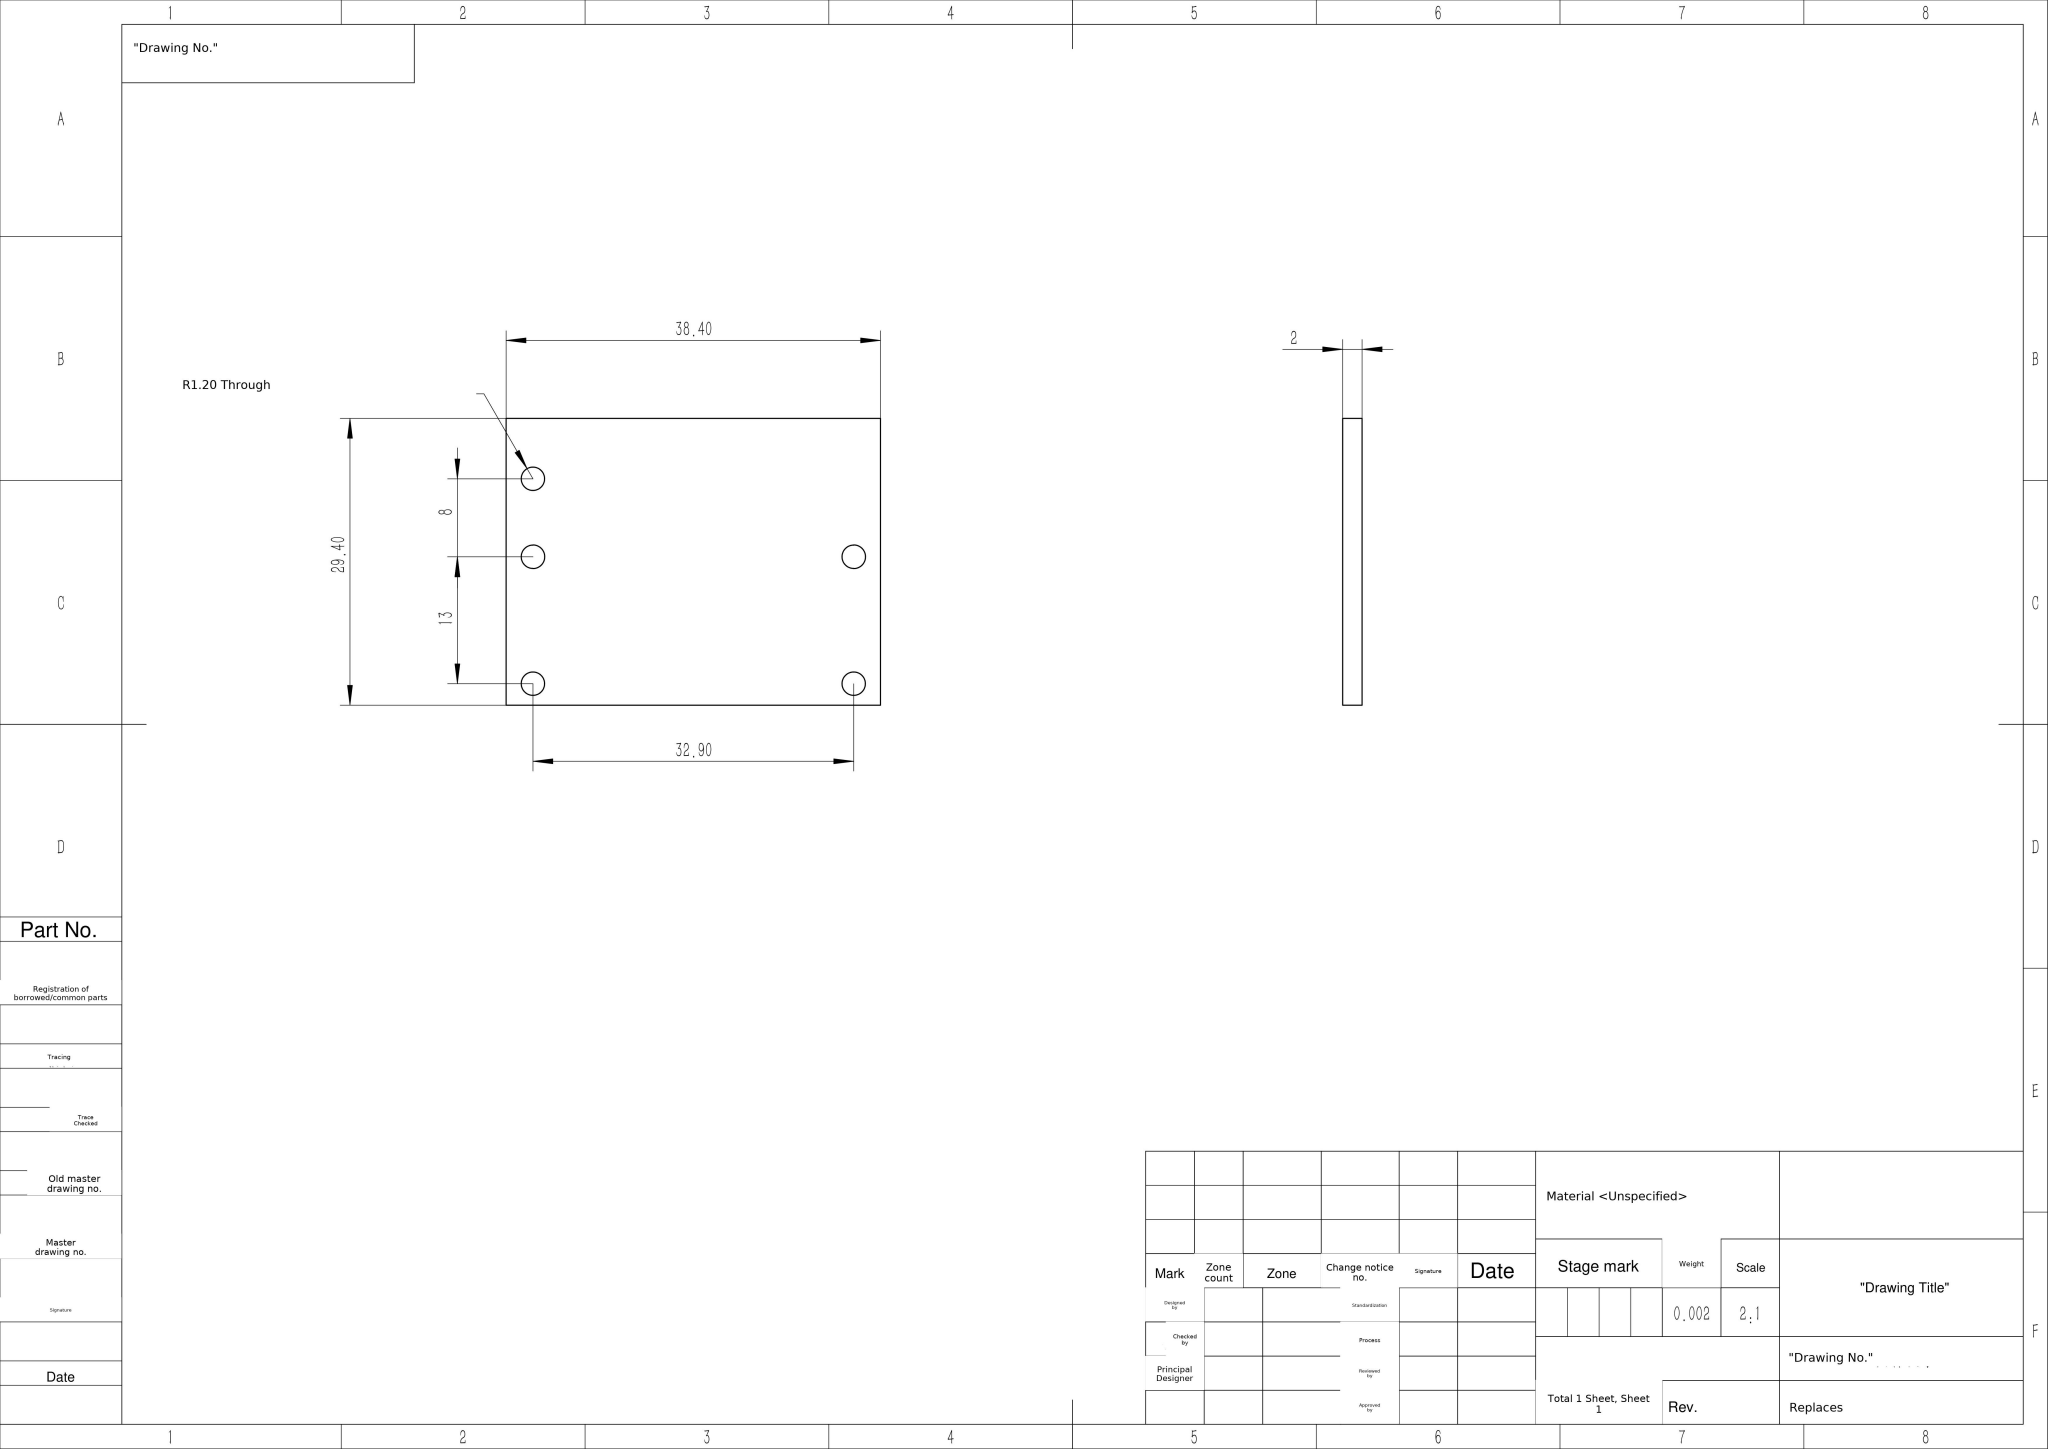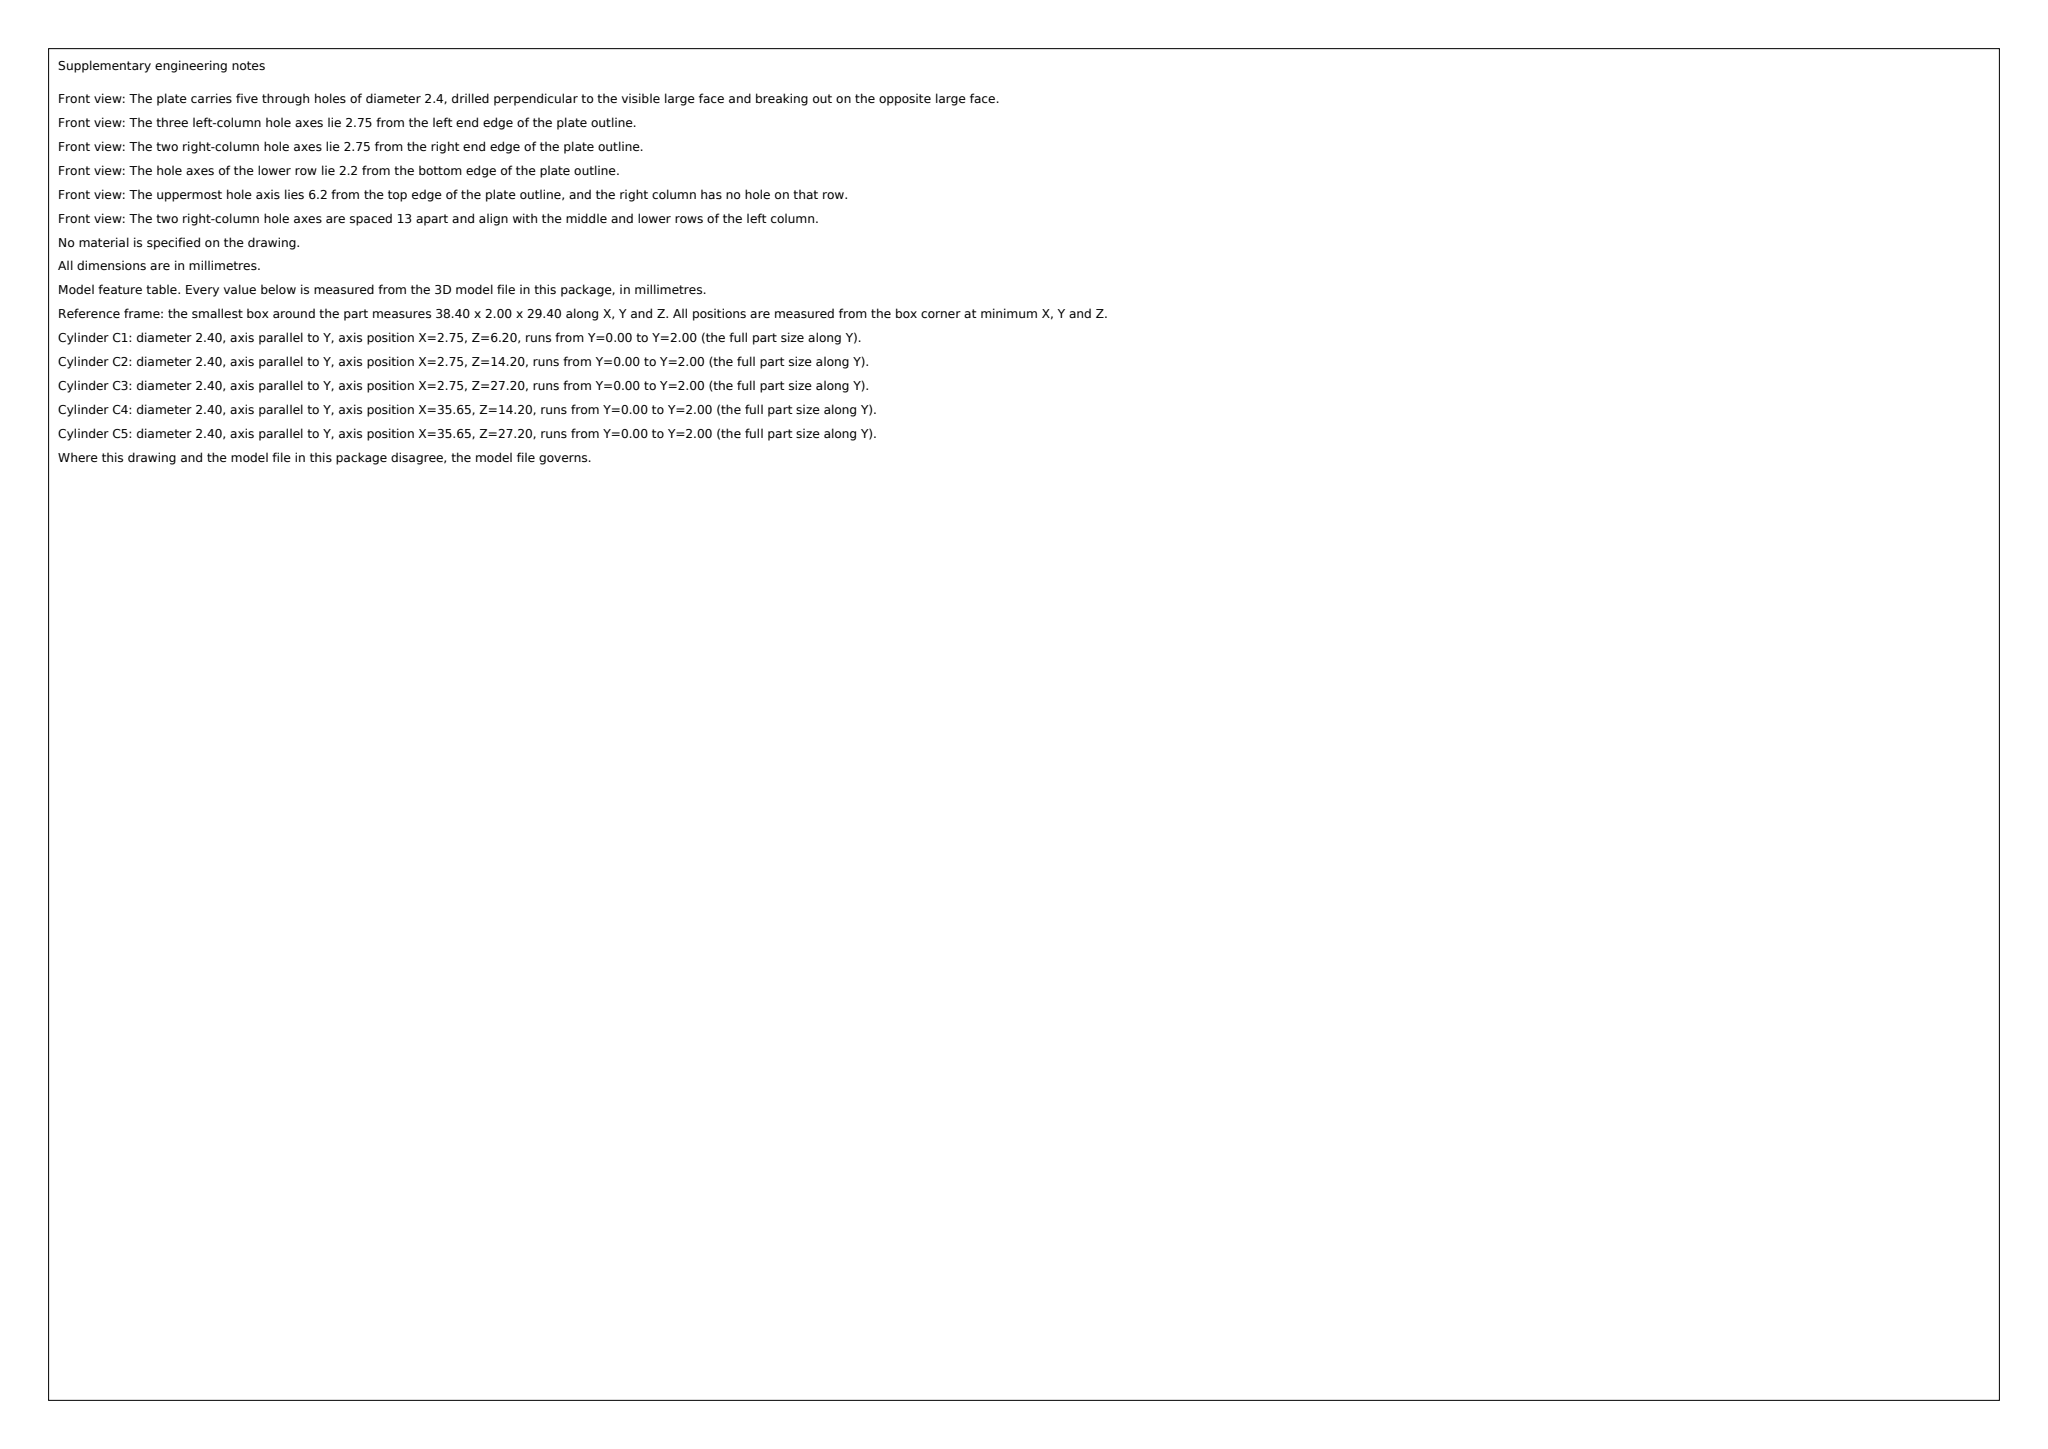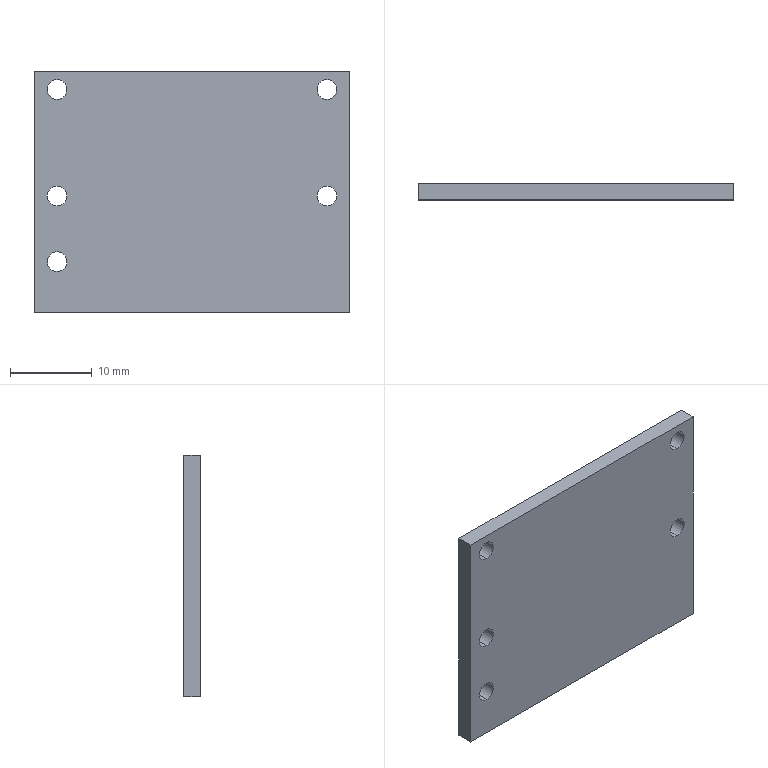Part | SolidWorks | mm | 1 solid | 16 faces | box 38.4 x 2 x 29.4 mm | volume 2213 mm3 | cylinder 10 | plane 6 | commonest cylinder face diameters 2.4 x10
Drawing notes:
TOP HOLE CL 2.2 FROM TOP EDGE; 8 & 13 TO LOWER HOLES | from the solid: Holes at z=27.2, 14.2, 6.2; plate height 29.4 -> 29.4-27.2=2.2
HOLE COL CL 2.75 FROM EA SIDE EDGE, 32.90 BETWEEN CL | from the solid: Hole x=2.75 and 35.65; bbox x=38.4 -> 38.4-35.65=2.75; 35.65-2.75=32.90
5X Ø2.4 THRU (R1.20) ALL HOLES | from the solid: Five cylinders dia 2.4, axis y, length 2.0 = full plate thickness 2.0
STEP:
#1=CARTESIAN_POINT('',(16.45,0.,-1.7));
#2=VERTEX_POINT('',#1);
#3=CARTESIAN_POINT('',(16.45,2.,-1.7));
#4=VERTEX_POINT('',#3);
#5=CARTESIAN_POINT('',(16.45,-0.001,-1.7));
#6=DIRECTION('',(0.,1.,0.));
#7=VECTOR('',#6,1000.);
#8=LINE('',#5,#7);
#9=EDGE_CURVE('',#2,#4,#8,.T.);
#10=ORIENTED_EDGE('',*,*,#9,.F.);
#11=CARTESIAN_POINT('',(16.45,0.,0.7));
#12=VERTEX_POINT('',#11);
#13=CARTESIAN_POINT('',(16.45,0.,-0.5));
#14=DIRECTION('',(0.,-1.,0.));
#15=DIRECTION('',(0.,0.,1.));
#16=AXIS2_PLACEMENT_3D('',#13,#14,#15);
#17=CIRCLE('',#16,1.2);
#18=EDGE_CURVE('',#2,#12,#17,.T.);
#19=ORIENTED_EDGE('',*,*,#18,.T.);
#20=CARTESIAN_POINT('',(16.45,2.,0.7));
#21=VERTEX_POINT('',#20);
#22=CARTESIAN_POINT('',(16.45,-0.001,0.7));
#23=DIRECTION('',(0.,1.,0.));
#24=VECTOR('',#23,1000.);
#25=LINE('',#22,#24);
#26=EDGE_CURVE('',#12,#21,#25,.T.);
#27=ORIENTED_EDGE('',*,*,#26,.T.);
#28=CARTESIAN_POINT('',(16.45,2.,-0.5));
#29=DIRECTION('',(0.,1.,0.));
#30=DIRECTION('',(0.,0.,1.));
#31=AXIS2_PLACEMENT_3D('',#28,#29,#30);
#32=CIRCLE('',#31,1.2);
#33=EDGE_CURVE('',#21,#4,#32,.T.);
#34=ORIENTED_EDGE('',*,*,#33,.T.);
#35=EDGE_LOOP('',(#10,#19,#27,#34));
#36=FACE_OUTER_BOUND('',#35,.T.);
#37=CARTESIAN_POINT('',(16.45,-0.001,-0.5));
#38=DIRECTION('',(0.,1.,0.));
#39=DIRECTION('',(0.,0.,1.));
#40=AXIS2_PLACEMENT_3D('',#37,#38,#39);
#41=CYLINDRICAL_SURFACE('',#40,1.2);
#42=ADVANCED_FACE('',(#36),#41,.F.);
#43=CARTESIAN_POINT('',(-16.45,0.,11.3));
#44=VERTEX_POINT('',#43);
#45=CARTESIAN_POINT('',(-16.45,2.,11.3));
#46=VERTEX_POINT('',#45);
#47=CARTESIAN_POINT('',(-16.45,-0.001,11.3));
#48=DIRECTION('',(0.,1.,0.));
#49=VECTOR('',#48,1000.);
#50=LINE('',#47,#49);
#51=EDGE_CURVE('',#44,#46,#50,.T.);
#52=ORIENTED_EDGE('',*,*,#51,.F.);
#53=CARTESIAN_POINT('',(-16.45,0.,13.7));
#54=VERTEX_POINT('',#53);
#55=CARTESIAN_POINT('',(-16.45,0.,12.5));
#56=DIRECTION('',(0.,-1.,0.));
#57=DIRECTION('',(0.,0.,1.));
#58=AXIS2_PLACEMENT_3D('',#55,#56,#57);
#59=CIRCLE('',#58,1.2);
#60=EDGE_CURVE('',#44,#54,#59,.T.);
#61=ORIENTED_EDGE('',*,*,#60,.T.);
#62=CARTESIAN_POINT('',(-16.45,2.,13.7));
#63=VERTEX_POINT('',#62);
#64=CARTESIAN_POINT('',(-16.45,-0.001,13.7));
#65=DIRECTION('',(0.,1.,0.));
#66=VECTOR('',#65,1000.);
#67=LINE('',#64,#66);
#68=EDGE_CURVE('',#54,#63,#67,.T.);
#69=ORIENTED_EDGE('',*,*,#68,.T.);
#70=CARTESIAN_POINT('',(-16.45,2.,12.5));
#71=DIRECTION('',(0.,1.,0.));
#72=DIRECTION('',(0.,0.,1.));
#73=AXIS2_PLACEMENT_3D('',#70,#71,#72);
#74=CIRCLE('',#73,1.2);
#75=EDGE_CURVE('',#63,#46,#74,.T.);
#76=ORIENTED_EDGE('',*,*,#75,.T.);
#77=EDGE_LOOP('',(#52,#61,#69,#76));
#78=FACE_OUTER_BOUND('',#77,.T.);
#79=CARTESIAN_POINT('',(-16.45,-0.001,12.5));
#80=DIRECTION('',(0.,1.,0.));
#81=DIRECTION('',(0.,0.,1.));
#82=AXIS2_PLACEMENT_3D('',#79,#80,#81);
#83=CYLINDRICAL_SURFACE('',#82,1.2);
#84=ADVANCED_FACE('',(#78),#83,.F.);
#85=CARTESIAN_POINT('',(-16.45,0.,-1.7));
#86=VERTEX_POINT('',#85);
#87=CARTESIAN_POINT('',(-16.45,2.,-1.7));
#88=VERTEX_POINT('',#87);
#89=CARTESIAN_POINT('',(-16.45,-0.001,-1.7));
#90=DIRECTION('',(0.,1.,0.));
#91=VECTOR('',#90,1000.);
#92=LINE('',#89,#91);
#93=EDGE_CURVE('',#86,#88,#92,.T.);
#94=ORIENTED_EDGE('',*,*,#93,.F.);
#95=CARTESIAN_POINT('',(-16.45,0.,0.7));
#96=VERTEX_POINT('',#95);
#97=CARTESIAN_POINT('',(-16.45,0.,-0.5));
#98=DIRECTION('',(0.,-1.,0.));
#99=DIRECTION('',(0.,0.,1.));
#100=AXIS2_PLACEMENT_3D('',#97,#98,#99);
#101=CIRCLE('',#100,1.2);
#102=EDGE_CURVE('',#86,#96,#101,.T.);
#103=ORIENTED_EDGE('',*,*,#102,.T.);
#104=CARTESIAN_POINT('',(-16.45,2.,0.7));
#105=VERTEX_POINT('',#104);
#106=CARTESIAN_POINT('',(-16.45,-0.001,0.7));
#107=DIRECTION('',(0.,1.,0.));
#108=VECTOR('',#107,1000.);
#109=LINE('',#106,#108);
#110=EDGE_CURVE('',#96,#105,#109,.T.);
#111=ORIENTED_EDGE('',*,*,#110,.T.);
#112=CARTESIAN_POINT('',(-16.45,2.,-0.5));
#113=DIRECTION('',(0.,1.,0.));
#114=DIRECTION('',(0.,0.,1.));
#115=AXIS2_PLACEMENT_3D('',#112,#113,#114);
#116=CIRCLE('',#115,1.2);
#117=EDGE_CURVE('',#105,#88,#116,.T.);
#118=ORIENTED_EDGE('',*,*,#117,.T.);
#119=EDGE_LOOP('',(#94,#103,#111,#118));
#120=FACE_OUTER_BOUND('',#119,.T.);
#121=CARTESIAN_POINT('',(-16.45,-0.001,-0.5));
#122=DIRECTION('',(0.,1.,0.));
#123=DIRECTION('',(0.,0.,1.));
#124=AXIS2_PLACEMENT_3D('',#121,#122,#123);
#125=CYLINDRICAL_SURFACE('',#124,1.2);
#126=ADVANCED_FACE('',(#120),#125,.F.);
#127=CARTESIAN_POINT('',(-16.45,0.,-9.7));
#128=VERTEX_POINT('',#127);
#129=CARTESIAN_POINT('',(-16.45,2.,-9.7));
#130=VERTEX_POINT('',#129);
#131=CARTESIAN_POINT('',(-16.45,-0.001,-9.7));
#132=DIRECTION('',(0.,1.,0.));
#133=VECTOR('',#132,1000.);
#134=LINE('',#131,#133);
#135=EDGE_CURVE('',#128,#130,#134,.T.);
#136=ORIENTED_EDGE('',*,*,#135,.F.);
#137=CARTESIAN_POINT('',(-16.45,0.,-7.3));
#138=VERTEX_POINT('',#137);
#139=CARTESIAN_POINT('',(-16.45,0.,-8.5));
#140=DIRECTION('',(0.,-1.,0.));
#141=DIRECTION('',(0.,0.,1.));
#142=AXIS2_PLACEMENT_3D('',#139,#140,#141);
#143=CIRCLE('',#142,1.2);
#144=EDGE_CURVE('',#128,#138,#143,.T.);
#145=ORIENTED_EDGE('',*,*,#144,.T.);
#146=CARTESIAN_POINT('',(-16.45,2.,-7.3));
#147=VERTEX_POINT('',#146);
#148=CARTESIAN_POINT('',(-16.45,-0.001,-7.3));
#149=DIRECTION('',(0.,1.,0.));
#150=VECTOR('',#149,1000.);
#151=LINE('',#148,#150);
#152=EDGE_CURVE('',#138,#147,#151,.T.);
#153=ORIENTED_EDGE('',*,*,#152,.T.);
#154=CARTESIAN_POINT('',(-16.45,2.,-8.5));
#155=DIRECTION('',(0.,1.,0.));
#156=DIRECTION('',(0.,0.,1.));
#157=AXIS2_PLACEMENT_3D('',#154,#155,#156);
#158=CIRCLE('',#157,1.2);
#159=EDGE_CURVE('',#147,#130,#158,.T.);
#160=ORIENTED_EDGE('',*,*,#159,.T.);
#161=EDGE_LOOP('',(#136,#145,#153,#160));
#162=FACE_OUTER_BOUND('',#161,.T.);
#163=CARTESIAN_POINT('',(-16.45,-0.001,-8.5));
#164=DIRECTION('',(0.,1.,0.));
#165=DIRECTION('',(0.,0.,1.));
#166=AXIS2_PLACEMENT_3D('',#163,#164,#165);
#167=CYLINDRICAL_SURFACE('',#166,1.2);
#168=ADVANCED_FACE('',(#162),#167,.F.);
#169=CARTESIAN_POINT('',(16.45,0.,11.3));
#170=VERTEX_POINT('',#169);
#171=CARTESIAN_POINT('',(16.45,2.,11.3));
#172=VERTEX_POINT('',#171);
#173=CARTESIAN_POINT('',(16.45,-0.001,11.3));
#174=DIRECTION('',(0.,1.,0.));
#175=VECTOR('',#174,1000.);
#176=LINE('',#173,#175);
#177=EDGE_CURVE('',#170,#172,#176,.T.);
#178=ORIENTED_EDGE('',*,*,#177,.F.);
#179=CARTESIAN_POINT('',(16.45,0.,13.7));
#180=VERTEX_POINT('',#179);
#181=CARTESIAN_POINT('',(16.45,0.,12.5));
#182=DIRECTION('',(0.,-1.,0.));
#183=DIRECTION('',(0.,0.,1.));
#184=AXIS2_PLACEMENT_3D('',#181,#182,#183);
#185=CIRCLE('',#184,1.2);
#186=EDGE_CURVE('',#170,#180,#185,.T.);
#187=ORIENTED_EDGE('',*,*,#186,.T.);
#188=CARTESIAN_POINT('',(16.45,2.,13.7));
#189=VERTEX_POINT('',#188);
#190=CARTESIAN_POINT('',(16.45,-0.001,13.7));
#191=DIRECTION('',(0.,1.,0.));
#192=VECTOR('',#191,1000.);
#193=LINE('',#190,#192);
#194=EDGE_CURVE('',#180,#189,#193,.T.);
#195=ORIENTED_EDGE('',*,*,#194,.T.);
#196=CARTESIAN_POINT('',(16.45,2.,12.5));
#197=DIRECTION('',(0.,1.,0.));
#198=DIRECTION('',(0.,0.,1.));
#199=AXIS2_PLACEMENT_3D('',#196,#197,#198);
#200=CIRCLE('',#199,1.2);
#201=EDGE_CURVE('',#189,#172,#200,.T.);
#202=ORIENTED_EDGE('',*,*,#201,.T.);
#203=EDGE_LOOP('',(#178,#187,#195,#202));
#204=FACE_OUTER_BOUND('',#203,.T.);
#205=CARTESIAN_POINT('',(16.45,-0.001,12.5));
#206=DIRECTION('',(0.,1.,0.));
#207=DIRECTION('',(0.,0.,1.));
#208=AXIS2_PLACEMENT_3D('',#205,#206,#207);
#209=CYLINDRICAL_SURFACE('',#208,1.2);
#210=ADVANCED_FACE('',(#204),#209,.F.);
#211=CARTESIAN_POINT('',(16.45,0.,12.5));
#212=DIRECTION('',(0.,-1.,0.));
#213=DIRECTION('',(0.,0.,1.));
#214=AXIS2_PLACEMENT_3D('',#211,#212,#213);
#215=CIRCLE('',#214,1.2);
#216=EDGE_CURVE('',#180,#170,#215,.T.);
#217=ORIENTED_EDGE('',*,*,#216,.F.);
#218=ORIENTED_EDGE('',*,*,#186,.F.);
#219=EDGE_LOOP('',(#217,#218));
#220=FACE_BOUND('',#219,.T.);
#221=CARTESIAN_POINT('',(-16.45,0.,-8.5));
#222=DIRECTION('',(0.,-1.,0.));
#223=DIRECTION('',(0.,0.,1.));
#224=AXIS2_PLACEMENT_3D('',#221,#222,#223);
#225=CIRCLE('',#224,1.2);
#226=EDGE_CURVE('',#138,#128,#225,.T.);
#227=ORIENTED_EDGE('',*,*,#226,.F.);
#228=ORIENTED_EDGE('',*,*,#144,.F.);
#229=EDGE_LOOP('',(#227,#228));
#230=FACE_BOUND('',#229,.T.);
#231=CARTESIAN_POINT('',(-16.45,0.,-0.5));
#232=DIRECTION('',(0.,-1.,0.));
#233=DIRECTION('',(0.,0.,1.));
#234=AXIS2_PLACEMENT_3D('',#231,#232,#233);
#235=CIRCLE('',#234,1.2);
#236=EDGE_CURVE('',#96,#86,#235,.T.);
#237=ORIENTED_EDGE('',*,*,#236,.F.);
#238=ORIENTED_EDGE('',*,*,#102,.F.);
#239=EDGE_LOOP('',(#237,#238));
#240=FACE_BOUND('',#239,.T.);
#241=CARTESIAN_POINT('',(-16.45,0.,12.5));
#242=DIRECTION('',(0.,-1.,0.));
#243=DIRECTION('',(0.,0.,1.));
#244=AXIS2_PLACEMENT_3D('',#241,#242,#243);
#245=CIRCLE('',#244,1.2);
#246=EDGE_CURVE('',#54,#44,#245,.T.);
#247=ORIENTED_EDGE('',*,*,#246,.F.);
#248=ORIENTED_EDGE('',*,*,#60,.F.);
#249=EDGE_LOOP('',(#247,#248));
#250=FACE_BOUND('',#249,.T.);
#251=CARTESIAN_POINT('',(16.45,0.,-0.5));
#252=DIRECTION('',(0.,-1.,0.));
#253=DIRECTION('',(0.,0.,1.));
#254=AXIS2_PLACEMENT_3D('',#251,#252,#253);
#255=CIRCLE('',#254,1.2);
#256=EDGE_CURVE('',#12,#2,#255,.T.);
#257=ORIENTED_EDGE('',*,*,#256,.F.);
#258=ORIENTED_EDGE('',*,*,#18,.F.);
#259=EDGE_LOOP('',(#257,#258));
#260=FACE_BOUND('',#259,.T.);
#261=CARTESIAN_POINT('',(19.2,0.,14.7));
#262=VERTEX_POINT('',#261);
#263=CARTESIAN_POINT('',(19.2,0.,-14.7));
#264=VERTEX_POINT('',#263);
#265=CARTESIAN_POINT('',(19.2,0.,-14.7));
#266=DIRECTION('',(0.,0.,-1.));
#267=VECTOR('',#266,1000.);
#268=LINE('',#265,#267);
#269=EDGE_CURVE('',#262,#264,#268,.T.);
#270=ORIENTED_EDGE('',*,*,#269,.F.);
#271=CARTESIAN_POINT('',(-19.2,0.,14.7));
#272=VERTEX_POINT('',#271);
#273=CARTESIAN_POINT('',(-19.2,0.,14.7));
#274=DIRECTION('',(1.,0.,0.));
#275=VECTOR('',#274,1000.);
#276=LINE('',#273,#275);
#277=EDGE_CURVE('',#272,#262,#276,.T.);
#278=ORIENTED_EDGE('',*,*,#277,.F.);
#279=CARTESIAN_POINT('',(-19.2,0.,-14.7));
#280=VERTEX_POINT('',#279);
#281=CARTESIAN_POINT('',(-19.2,0.,-14.7));
#282=DIRECTION('',(0.,0.,1.));
#283=VECTOR('',#282,1000.);
#284=LINE('',#281,#283);
#285=EDGE_CURVE('',#280,#272,#284,.T.);
#286=ORIENTED_EDGE('',*,*,#285,.F.);
#287=CARTESIAN_POINT('',(-19.2,0.,-14.7));
#288=DIRECTION('',(-1.,0.,0.));
#289=VECTOR('',#288,1000.);
#290=LINE('',#287,#289);
#291=EDGE_CURVE('',#264,#280,#290,.T.);
#292=ORIENTED_EDGE('',*,*,#291,.F.);
#293=EDGE_LOOP('',(#270,#278,#286,#292));
#294=FACE_OUTER_BOUND('',#293,.T.);
#295=CARTESIAN_POINT('',(0.,0.,0.));
#296=DIRECTION('',(0.,1.,0.));
#297=DIRECTION('',(1.,0.,0.));
#298=AXIS2_PLACEMENT_3D('',#295,#296,#297);
#299=PLANE('',#298);
#300=ADVANCED_FACE('',(#220,#230,#240,#250,#260,#294),#299,.F.);
#301=ORIENTED_EDGE('',*,*,#201,.F.);
#302=CARTESIAN_POINT('',(16.45,2.,12.5));
#303=DIRECTION('',(0.,1.,0.));
#304=DIRECTION('',(0.,0.,1.));
#305=AXIS2_PLACEMENT_3D('',#302,#303,#304);
#306=CIRCLE('',#305,1.2);
#307=EDGE_CURVE('',#172,#189,#306,.T.);
#308=ORIENTED_EDGE('',*,*,#307,.F.);
#309=EDGE_LOOP('',(#301,#308));
#310=FACE_BOUND('',#309,.T.);
#311=ORIENTED_EDGE('',*,*,#159,.F.);
#312=CARTESIAN_POINT('',(-16.45,2.,-8.5));
#313=DIRECTION('',(0.,1.,0.));
#314=DIRECTION('',(0.,0.,1.));
#315=AXIS2_PLACEMENT_3D('',#312,#313,#314);
#316=CIRCLE('',#315,1.2);
#317=EDGE_CURVE('',#130,#147,#316,.T.);
#318=ORIENTED_EDGE('',*,*,#317,.F.);
#319=EDGE_LOOP('',(#311,#318));
#320=FACE_BOUND('',#319,.T.);
#321=ORIENTED_EDGE('',*,*,#117,.F.);
#322=CARTESIAN_POINT('',(-16.45,2.,-0.5));
#323=DIRECTION('',(0.,1.,0.));
#324=DIRECTION('',(0.,0.,1.));
#325=AXIS2_PLACEMENT_3D('',#322,#323,#324);
#326=CIRCLE('',#325,1.2);
#327=EDGE_CURVE('',#88,#105,#326,.T.);
#328=ORIENTED_EDGE('',*,*,#327,.F.);
#329=EDGE_LOOP('',(#321,#328));
#330=FACE_BOUND('',#329,.T.);
#331=ORIENTED_EDGE('',*,*,#75,.F.);
#332=CARTESIAN_POINT('',(-16.45,2.,12.5));
#333=DIRECTION('',(0.,1.,0.));
#334=DIRECTION('',(0.,0.,1.));
#335=AXIS2_PLACEMENT_3D('',#332,#333,#334);
#336=CIRCLE('',#335,1.2);
#337=EDGE_CURVE('',#46,#63,#336,.T.);
#338=ORIENTED_EDGE('',*,*,#337,.F.);
#339=EDGE_LOOP('',(#331,#338));
#340=FACE_BOUND('',#339,.T.);
#341=ORIENTED_EDGE('',*,*,#33,.F.);
#342=CARTESIAN_POINT('',(16.45,2.,-0.5));
#343=DIRECTION('',(0.,1.,0.));
#344=DIRECTION('',(0.,0.,1.));
#345=AXIS2_PLACEMENT_3D('',#342,#343,#344);
#346=CIRCLE('',#345,1.2);
#347=EDGE_CURVE('',#4,#21,#346,.T.);
#348=ORIENTED_EDGE('',*,*,#347,.F.);
#349=EDGE_LOOP('',(#341,#348));
#350=FACE_BOUND('',#349,.T.);
#351=CARTESIAN_POINT('',(19.2,2.,14.7));
#352=VERTEX_POINT('',#351);
#353=CARTESIAN_POINT('',(19.2,2.,-14.7));
#354=VERTEX_POINT('',#353);
#355=CARTESIAN_POINT('',(19.2,2.,-14.7));
#356=DIRECTION('',(0.,0.,-1.));
#357=VECTOR('',#356,1000.);
#358=LINE('',#355,#357);
#359=EDGE_CURVE('',#352,#354,#358,.T.);
#360=ORIENTED_EDGE('',*,*,#359,.T.);
#361=CARTESIAN_POINT('',(-19.2,2.,-14.7));
#362=VERTEX_POINT('',#361);
#363=CARTESIAN_POINT('',(-19.2,2.,-14.7));
#364=DIRECTION('',(-1.,0.,0.));
#365=VECTOR('',#364,1000.);
#366=LINE('',#363,#365);
#367=EDGE_CURVE('',#354,#362,#366,.T.);
#368=ORIENTED_EDGE('',*,*,#367,.T.);
#369=CARTESIAN_POINT('',(-19.2,2.,14.7));
#370=VERTEX_POINT('',#369);
#371=CARTESIAN_POINT('',(-19.2,2.,-14.7));
#372=DIRECTION('',(0.,0.,1.));
#373=VECTOR('',#372,1000.);
#374=LINE('',#371,#373);
#375=EDGE_CURVE('',#362,#370,#374,.T.);
#376=ORIENTED_EDGE('',*,*,#375,.T.);
#377=CARTESIAN_POINT('',(-19.2,2.,14.7));
#378=DIRECTION('',(1.,0.,0.));
#379=VECTOR('',#378,1000.);
#380=LINE('',#377,#379);
#381=EDGE_CURVE('',#370,#352,#380,.T.);
#382=ORIENTED_EDGE('',*,*,#381,.T.);
#383=EDGE_LOOP('',(#360,#368,#376,#382));
#384=FACE_OUTER_BOUND('',#383,.T.);
#385=CARTESIAN_POINT('',(0.,2.,0.));
#386=DIRECTION('',(0.,1.,0.));
#387=DIRECTION('',(1.,0.,0.));
#388=AXIS2_PLACEMENT_3D('',#385,#386,#387);
#389=PLANE('',#388);
#390=ADVANCED_FACE('',(#310,#320,#330,#340,#350,#384),#389,.T.);
#391=ORIENTED_EDGE('',*,*,#277,.T.);
#392=CARTESIAN_POINT('',(19.2,2.,14.7));
#393=DIRECTION('',(0.,-1.,0.));
#394=VECTOR('',#393,1000.);
#395=LINE('',#392,#394);
#396=EDGE_CURVE('',#352,#262,#395,.T.);
#397=ORIENTED_EDGE('',*,*,#396,.F.);
#398=ORIENTED_EDGE('',*,*,#381,.F.);
#399=CARTESIAN_POINT('',(-19.2,2.,14.7));
#400=DIRECTION('',(0.,-1.,0.));
#401=VECTOR('',#400,1000.);
#402=LINE('',#399,#401);
#403=EDGE_CURVE('',#370,#272,#402,.T.);
#404=ORIENTED_EDGE('',*,*,#403,.T.);
#405=EDGE_LOOP('',(#391,#397,#398,#404));
#406=FACE_OUTER_BOUND('',#405,.T.);
#407=CARTESIAN_POINT('',(-19.2,2.,14.7));
#408=DIRECTION('',(0.,0.,-1.));
#409=DIRECTION('',(0.,-1.,0.));
#410=AXIS2_PLACEMENT_3D('',#407,#408,#409);
#411=PLANE('',#410);
#412=ADVANCED_FACE('',(#406),#411,.F.);
#413=ORIENTED_EDGE('',*,*,#285,.T.);
#414=ORIENTED_EDGE('',*,*,#403,.F.);
#415=ORIENTED_EDGE('',*,*,#375,.F.);
#416=CARTESIAN_POINT('',(-19.2,2.,-14.7));
#417=DIRECTION('',(0.,-1.,0.));
#418=VECTOR('',#417,1000.);
#419=LINE('',#416,#418);
#420=EDGE_CURVE('',#362,#280,#419,.T.);
#421=ORIENTED_EDGE('',*,*,#420,.T.);
#422=EDGE_LOOP('',(#413,#414,#415,#421));
#423=FACE_OUTER_BOUND('',#422,.T.);
#424=CARTESIAN_POINT('',(-19.2,2.,-14.7));
#425=DIRECTION('',(1.,0.,0.));
#426=DIRECTION('',(0.,1.,0.));
#427=AXIS2_PLACEMENT_3D('',#424,#425,#426);
#428=PLANE('',#427);
#429=ADVANCED_FACE('',(#423),#428,.F.);
#430=ORIENTED_EDGE('',*,*,#291,.T.);
#431=ORIENTED_EDGE('',*,*,#420,.F.);
#432=ORIENTED_EDGE('',*,*,#367,.F.);
#433=CARTESIAN_POINT('',(19.2,2.,-14.7));
#434=DIRECTION('',(0.,-1.,0.));
#435=VECTOR('',#434,1000.);
#436=LINE('',#433,#435);
#437=EDGE_CURVE('',#354,#264,#436,.T.);
#438=ORIENTED_EDGE('',*,*,#437,.T.);
#439=EDGE_LOOP('',(#430,#431,#432,#438));
#440=FACE_OUTER_BOUND('',#439,.T.);
#441=CARTESIAN_POINT('',(-19.2,2.,-14.7));
#442=DIRECTION('',(0.,0.,1.));
#443=DIRECTION('',(1.,0.,0.));
#444=AXIS2_PLACEMENT_3D('',#441,#442,#443);
#445=PLANE('',#444);
#446=ADVANCED_FACE('',(#440),#445,.F.);
#447=ORIENTED_EDGE('',*,*,#269,.T.);
#448=ORIENTED_EDGE('',*,*,#437,.F.);
#449=ORIENTED_EDGE('',*,*,#359,.F.);
#450=ORIENTED_EDGE('',*,*,#396,.T.);
#451=EDGE_LOOP('',(#447,#448,#449,#450));
#452=FACE_OUTER_BOUND('',#451,.T.);
#453=CARTESIAN_POINT('',(19.2,2.,-14.7));
#454=DIRECTION('',(-1.,0.,0.));
#455=DIRECTION('',(0.,0.,1.));
#456=AXIS2_PLACEMENT_3D('',#453,#454,#455);
#457=PLANE('',#456);
#458=ADVANCED_FACE('',(#452),#457,.F.);
#459=ORIENTED_EDGE('',*,*,#216,.T.);
#460=ORIENTED_EDGE('',*,*,#177,.T.);
#461=ORIENTED_EDGE('',*,*,#307,.T.);
#462=ORIENTED_EDGE('',*,*,#194,.F.);
#463=EDGE_LOOP('',(#459,#460,#461,#462));
#464=FACE_OUTER_BOUND('',#463,.T.);
#465=CARTESIAN_POINT('',(16.45,-0.001,12.5));
#466=DIRECTION('',(0.,1.,0.));
#467=DIRECTION('',(0.,0.,1.));
#468=AXIS2_PLACEMENT_3D('',#465,#466,#467);
#469=CYLINDRICAL_SURFACE('',#468,1.2);
#470=ADVANCED_FACE('',(#464),#469,.F.);
#471=ORIENTED_EDGE('',*,*,#226,.T.);
#472=ORIENTED_EDGE('',*,*,#135,.T.);
#473=ORIENTED_EDGE('',*,*,#317,.T.);
#474=ORIENTED_EDGE('',*,*,#152,.F.);
#475=EDGE_LOOP('',(#471,#472,#473,#474));
#476=FACE_OUTER_BOUND('',#475,.T.);
#477=CARTESIAN_POINT('',(-16.45,-0.001,-8.5));
#478=DIRECTION('',(0.,1.,0.));
#479=DIRECTION('',(0.,0.,1.));
#480=AXIS2_PLACEMENT_3D('',#477,#478,#479);
#481=CYLINDRICAL_SURFACE('',#480,1.2);
#482=ADVANCED_FACE('',(#476),#481,.F.);
#483=ORIENTED_EDGE('',*,*,#236,.T.);
#484=ORIENTED_EDGE('',*,*,#93,.T.);
#485=ORIENTED_EDGE('',*,*,#327,.T.);
#486=ORIENTED_EDGE('',*,*,#110,.F.);
#487=EDGE_LOOP('',(#483,#484,#485,#486));
#488=FACE_OUTER_BOUND('',#487,.T.);
#489=CARTESIAN_POINT('',(-16.45,-0.001,-0.5));
#490=DIRECTION('',(0.,1.,0.));
#491=DIRECTION('',(0.,0.,1.));
#492=AXIS2_PLACEMENT_3D('',#489,#490,#491);
#493=CYLINDRICAL_SURFACE('',#492,1.2);
#494=ADVANCED_FACE('',(#488),#493,.F.);
#495=ORIENTED_EDGE('',*,*,#246,.T.);
#496=ORIENTED_EDGE('',*,*,#51,.T.);
#497=ORIENTED_EDGE('',*,*,#337,.T.);
#498=ORIENTED_EDGE('',*,*,#68,.F.);
#499=EDGE_LOOP('',(#495,#496,#497,#498));
#500=FACE_OUTER_BOUND('',#499,.T.);
#501=CARTESIAN_POINT('',(-16.45,-0.001,12.5));
#502=DIRECTION('',(0.,1.,0.));
#503=DIRECTION('',(0.,0.,1.));
#504=AXIS2_PLACEMENT_3D('',#501,#502,#503);
#505=CYLINDRICAL_SURFACE('',#504,1.2);
#506=ADVANCED_FACE('',(#500),#505,.F.);
#507=ORIENTED_EDGE('',*,*,#256,.T.);
#508=ORIENTED_EDGE('',*,*,#9,.T.);
#509=ORIENTED_EDGE('',*,*,#347,.T.);
#510=ORIENTED_EDGE('',*,*,#26,.F.);
#511=EDGE_LOOP('',(#507,#508,#509,#510));
#512=FACE_OUTER_BOUND('',#511,.T.);
#513=CARTESIAN_POINT('',(16.45,-0.001,-0.5));
#514=DIRECTION('',(0.,1.,0.));
#515=DIRECTION('',(0.,0.,1.));
#516=AXIS2_PLACEMENT_3D('',#513,#514,#515);
#517=CYLINDRICAL_SURFACE('',#516,1.2);
#518=ADVANCED_FACE('',(#512),#517,.F.);
#519=CLOSED_SHELL('',(#42,#84,#126,#168,#210,#300,#390,#412,#429,#446,#458,#470,#482,#494,#506,#518));
#520=MANIFOLD_SOLID_BREP('',#519);
#521=CARTESIAN_POINT('',(0.,0.,0.));
#522=DIRECTION('',(0.,0.,1.));
#523=DIRECTION('',(1.,0.,0.));
#524=AXIS2_PLACEMENT_3D('',#521,#522,#523);
#525=(LENGTH_UNIT()NAMED_UNIT(*)SI_UNIT(.MILLI.,.METRE.));
#526=UNCERTAINTY_MEASURE_WITH_UNIT(LENGTH_MEASURE(0.00001),#525,'','');
#527=(NAMED_UNIT(*)PLANE_ANGLE_UNIT()SI_UNIT($,.RADIAN.));
#528=(NAMED_UNIT(*)SI_UNIT($,.STERADIAN.)SOLID_ANGLE_UNIT());
#529=(GEOMETRIC_REPRESENTATION_CONTEXT(3)GLOBAL_UNCERTAINTY_ASSIGNED_CONTEXT((#526))GLOBAL_UNIT_ASSIGNED_CONTEXT((#525,#527,#528))REPRESENTATION_CONTEXT('',''));
#530=ADVANCED_BREP_SHAPE_REPRESENTATION('',(#520,#524),#529);